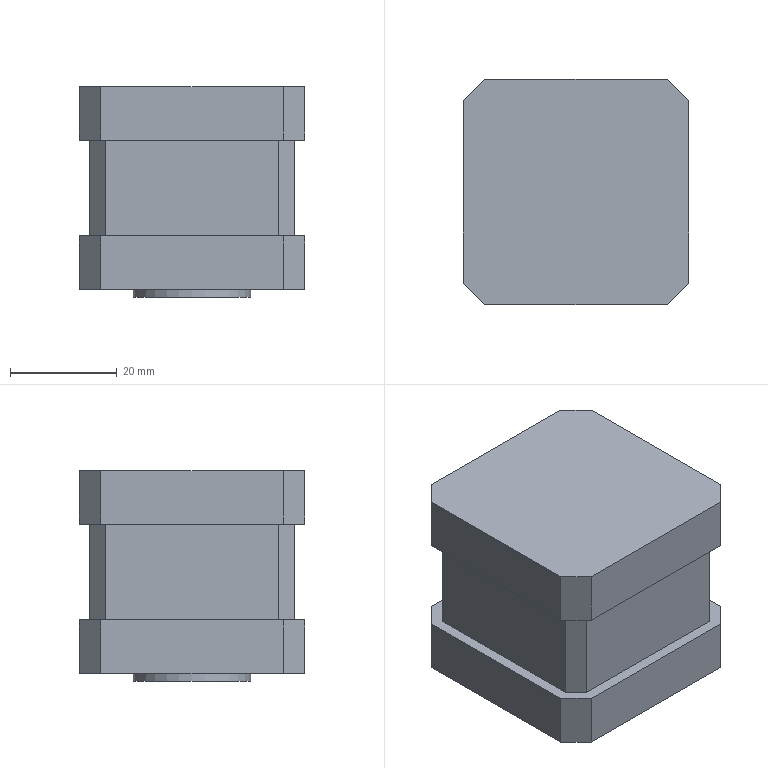Component | NX | SIMMOTOR | 1 solid | 44 faces | volume 60927 mm3 | plane 30 | cone 8 | cylinder 6 | commonest cylinder face diameters 3 x4 22 x1 8 x1